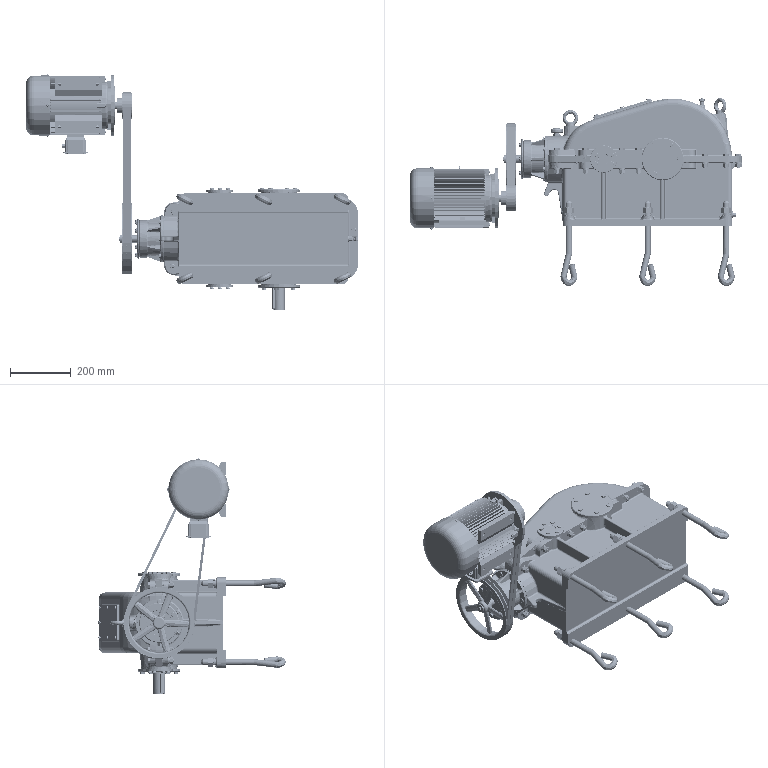Assembly | SolidWorks | mm | 166 component files | 167 solids | 7036 faces | box 1096.96 x 620.43 x 778.46 mm | volume 26160127 mm3 | plane 2138 | cone 2016 | cylinder 1637 | spline 832 | torus 356 | sphere 57 | commonest cylinder face diameters 8 x245 20 x128 324 x107 310.492 x106 6 x100 13.5 x78 10 x76 12 x74
Bill of materials:
BevelGear24_2.5 | 1 |  | Bevel-type pinion: a conical toothed body with a plain cylindrical hub on its back side and a through bore with one keyway.
BevelGear82_2.51 | 1 |  | Large, flat bevel-type gear: a wide disc with many fine teeth on a conical outer face, a flat central face, a small hub boss on the back and a keyed bore.
BreatherCap | 1 | Q235-A | Turned part with a mushroom-shaped head: a large domed, chamfered round head, a waisted neck, a hex section and a cylindrical spigot with a small axial bore.
Bushing0718 | 1 |  | Flanged, hollow, axisymmetric hub or housing: a large bolt flange between a short wide collar on one side and a long cylindrical barrel on the other, joined by gusset ribs, with a central through bore.
CylindricalGear106_3 | 1 |  | Spur gear with straight teeth: a thin, wide disc with many fine teeth, a recessed web with six lightening/through holes, a raised central hub and a keyed bore.
CylindricalGear24_3 | 1 |  | Spur gear with a long face width: straight teeth along a long cylindrical body and a through bore with one keyway.
Default | 1 |  | Envelope looks like a foot- and flange-mounted rotating machine, similar to an electric motor: a finned cylindrical body, a domed rear cover, a mounting foot, a front flange and a protruding plain shaft.
Gasket | 2 |  | Plain flat washer-like ring: a thin annular disc with a central round hole and parallel flat faces.
GB_T10708.3-1989TypeBRubberDustSealFB20_35_7 | 1 |  | Stepped ring: a rectangular-section annulus with a smaller-diameter, chamfered or tapered lip on one face, and a thin wall relative to its diameter.
GB_T10708.3-1989TypeBRubberDustSealFB45_65_8 | 1 |  | Wide, thin annular ring with a conical (tapered) inner bore and a short tapered shoulder below a flat-sided main band.
GB_T117-2000[TaperPin8_30] | 2 |  | Solid cylindrical pin with slightly domed/crowned ends on both sides; resembles a dowel-type pin.
Default | 4 |  | Rolling-element bearing-like assembly: concentric outer and inner rings with a single row of rolling elements between them; the inner ring sticks out axially past the outer ring on one side.
Default | 2 |  | Rolling-element bearing-like assembly with thinner section: outer and inner rings with one row of rolling elements; the inner ring sticks out axially on one side; larger bore relative to outer diameter than unnamed part.
GB_T41-2000HexNutType1C-gradeM20 | 6 |  | Hexagonal prism with a plain round through-bore, chamfered corners on both end faces; nut-like shape.
GB_T5780-2016[HexHeadBoltGradeCM12_80] | 8 |  | Hex-head bolt-like part with a long, plain cylindrical shank and chamfered tip.
GB_T5781-2000[HexHeadBoltFullThreadGradeCM12_40] | 5 |  | Hex-head bolt-like part with a medium-length plain cylindrical shank and chamfered tip.
GB_T5781-2000[HexHeadBoltFullThreadGradeCM6_16] | 8 |  | Short hex-head bolt-like part with a plain cylindrical shank, small fillet under the head and chamfered tip.
GB_T5781-2000[HexHeadBoltFullThreadGradeCM8_16] | 30 |  | Short hex-head bolt-like part with a plain shank, about 2x head width in length, and a chamfered tip.
GB_T5781-2000[HexHeadBoltFullThreadGradeCM8_20] | 6 |  | Short hex-head bolt-like part with a plain cylindrical shank and chamfered tip.
GB_T5781-2000HexHeadBoltFullThreadC-gradeM10_30 | 1 |  | Hex-head bolt-like part: hexagonal head with chamfered top edges, a thin cylindrical shoulder under the head, and a smooth cylindrical shank with a chamfered tip.
GB_T5781-2000HexHeadBoltFullThreadC-gradeM8_25 | 1 |  | Hex-head bolt-like part with a round washer-face flange under the head and a smooth cylindrical shank ending in a chamfered tip.
GB_T6170-2000[Type1HexNutGradeAAndBM12] | 13 |  | Hexagonal nut-like body with a central through bore and chamfered corners on both faces.
GB_T825-1988[LiftingEyeBoltM20] | 2 |  | Eye-shaped part: a toroidal ring loop on a cylindrical collar, with a plain cylindrical shank coming out of the collar.
GB_T93-1987[StandardSpringWasher(Assembly)12] | 13 |  | Flat annular ring with one narrow radial cut through the ring; the ends sit in the same plane.
GB_T93-1987StandardSpringWasher(Part)20_10 | 6 |  | Split annular ring with a rectangular section, twisted into one helical turn so the cut ends are offset along the axis; spring-lock-washer-like shape.
GB_T95-2002[FlatWasherGradeC12] | 13 |  | Plain flat annular disc (washer-like) with square edges and a central round hole.
GB_T97.2-1985FlatWasherChamferedTypeA-grade20_3 | 6 |  | Thin flat annular disc with a central round hole and a small chamfer on one outer edge.
HighSpeedAxisEndCoverA | 1 |  | Thin circular flange plate with six evenly spaced through-holes on a bolt circle and a central raised stepped cylindrical boss with a through-bore.
InputAxis | 1 |  | Stepped cylindrical shaft with several diameter sections, a larger central section, and one end face with a conical centre recess and a small slot or notch at the edge.
IntermediateAxis | 1 |  | Stepped cylindrical shaft with a thin raised collar ring partway along its length and a small notch at one end.
JB_ZQ4363-2006AnchorBoltTypeA20_630 | 6 |  | Bent round wire with a tight teardrop-shaped eye loop at one end, a short angled leg, and a long straight leg with a chamfered tip; cotter-pin-like or hook-like form.
JB_ZQ4450-1997[ExternalHexPlugM12_1.25] | 1 |  | Plug-like part: external hex drive, thin circular flange, undercut groove, and a chamfered cylindrical pilot/shank.
Key12-8-70 | 1 |  | Rectangular bar with fully rounded ends and slightly chamfered edges; parallel-key-like prism.
Key16-10-63 | 1 |  | Solid bar with rounded ends: a straight prism whose outline is a rectangle with two semicircular ends, with small chamfers on the edges. Moderately elongated, roughly 3.5:1 length to width in the rendered view.
Key6-6-25 | 1 |  | Short, stocky bar with rounded ends: a stadium-outline prism with chamfered edges, about 2.4:1 length to width, with height close to width.
Key6-6-32 | 1 |  | Bar with rounded ends: a stadium-outline prism with chamfered edges, about 3.2:1 length to width.
Key8-7-28 | 1 |  | Bar with rounded ends: a stadium-outline prism with chamfered edges, about 2.8:1 length to width, with a near-square cross-section.
Key8-7-40 | 1 |  | Long, slender bar with rounded ends: a stadium-outline prism with chamfered edges, about 5:1 length to width.
Key8-7-70 | 1 |  | Very slender bar with rounded ends: a stadium-outline prism with chamfered edges, about 7:1 length to width.
MachineBase | 1 |  | Open-top, box-shaped housing body. A rectangular wall shell is divided into compartments by internal ribs. The top has a perimeter flange interrupted by two semicircular cut-outs of different sizes, each with a bolt-hole pattern on the boss face. There are flanged ends with holes, extra holes on the side walls, and a hook-like lug on each end.
MachineCover | 1 |  | Hollow cover shell with an arched, sloping crown on top of a flat perimeter flange. The flange has two semicircular cut-outs of different sizes with small hole patterns, plus many perimeter holes. The top face has a rectangular opening ringed by small holes, and there are bosses or side protrusions on an end wall.
OilGauge | 1 |  | Long, thin, straight cylindrical rod or tube with a stepped head at one end. The head has a knurled or toothed outer cap, with concentric raised rings on its end face.
OutputAxis0717 | 1 |  | Stepped cylindrical shaft. Several diameters step down along its length, there is a thin raised collar near the middle, and keyway-like slots are cut into two of the diameter sections.
OutputAxisEndCover2-0717 | 1 |  | Solid circular cover disc with a chamfered outer edge and six through holes evenly spaced on a bolt circle. One face has a stepped, two-diameter spigot, with no central bore.
OutputAxisEndCover2-0718 | 1 |  | Flanged ring with a large central through bore. A wide chamfered base flange carries six evenly spaced through holes. A stepped intermediate ring and a raised cylindrical boss surround the bore.
SecondaryEndCover | 2 |  | Round, flat flange-like disc with six holes evenly spaced on a bolt circle. A circular feature sits at the center of the top face, and the underside steps down through a slightly smaller shoulder to a smaller cylindrical spigot.
SightHoleCoverA | 1 |  | Thin, flat rectangular plate with rounded corners and eight small round through holes around its edges.
V-beltL459x2 | 1 | Rubber | Closed teardrop- or pear-shaped loop made of a thin band, with a large rounded end, a small rounded end and two straight sides that taper between them. Edge views show two parallel bands side by side with a narrow gap between them.
A | 1 | Plain Carbon Steel | Spoked wheel with a twin-groove rim, resembling a two-groove V-belt pulley.
V-beltSmallSolidWheel86x24.075x48 | 1 | Plain Carbon Steel | Pulley-like body of revolution with two V-shaped circumferential grooves and a cylindrical hub on one side. A central through bore has a single rectangular keyway.
Mates:
1. concentric | OutputAxis0717-1 face at (-30, 0, 58.75) dir (0, 0, -1) r 27.5 | CylindricalGear106_3-1 face at (-30, 0, 35.75) dir (0, 0, 1) r 44
2. concentric | IntermediateAxis-1 face at (-225, 0, -13.099) dir (0, 0, 1) r 15 | CylindricalGear24_3-1 face at (-225, 0, 76.901) dir (0, 0, -1) r 15
3. concentric | IntermediateAxis-1 face at (-225, 0, -56.099) dir (0, 0, 1) r 15 | BevelGear82_2.51-1 face at (-225, 0, -6.098) dir (0, 0, -1) r 15
4. coincident | IntermediateAxis-1 face at (-225, 0, -23.099) dir (0, 0, -1) | BevelGear82_2.51-1 face at (-271.987, 53.409, -23.099) dir (0, 0, 1)
5. coincident | BevelGear82_2.51-1 sketch point at (-225, 0, 0) dir (1, 0, 0) | BevelGear24_2.5-1 sketch point at (-225, 0, 0) dir (1, 0, 0)
6. concentric | MachineBase-1 face at (200.001, 0, 0) dir (-1, 0, 0) r 54 | BevelGear24_2.5-1 face at (-357.363, 0, 0) dir (1, 0, 0) r 16
7. perpendicular | BevelGear82_2.51-1 face at (-227.438, 2.771, -56.098) dir (0, 0, -1) | BevelGear24_2.5-1 face at (-330.363, 2.308, -2.88) dir (-1, 0, 0)
8. concentric | InputAxis-1 face at (-297.364, 0, 0) dir (-1, 0, 0) r 10 | BevelGear24_2.5-1 face at (-357.363, 0, 0) dir (1, 0, 0) r 16
9. coincident | InputAxis-1 face at (-297.364, 0, 0) dir (1, 0, 0) | BevelGear24_2.5-1 face at (-297.364, 11.819, -14.749) dir (1, 0, 0)
10. concentric | MachineBase-1 face at (200.001, 0, 0) dir (-1, 0, 0) r 54 | Bushing0718-1 face at (-490, 0, 0) dir (-1, 0, 0) r 54
11. concentric | MachineBase-1 face at (-225, 0, -147) dir (0, 0, 1) r 26 | IntermediateAxis-1 face at (-225, 0, 61.901) dir (0, 0, 1) r 12.5
12. coincident | MachineBase-1 face at (-410, 0, 0) dir (-1, 0, 0) | Bushing0718-1 face at (-410, 38.5, -66.684) dir (1, 0, 0)
13. concentric | MachineBase-1 face at (-225, 0, -147) dir (0, 0, 1) r 26 | IntermediateAxis-1 face at (-225, 0, 61.901) dir (0, 0, 1) r 12.5
14. concentric | MachineBase-1 face at (-30, 0, -147) dir (0, 0, 1) r 45 | OutputAxis0717-1 face at (-30, 0, 107.25) dir (0, 0, -1) r 25
15. concentric | OutputAxis0717-1 face at (-30, 0, 107.25) dir (0, 0, -1) r 25 | GB_T297-94TaperedRollerBearing30210-0717-1 face at (-30, 0, 109) dir (0, 0, 1) r 25
16. coincident | OutputAxis0717-1 face at (-30, 0, 107.25) dir (0, 0, 1) | GB_T297-94TaperedRollerBearing30210-0717-1 face at (-27.138, 32.397, 107.25) dir (0, 0, 1)
17. concentric | OutputAxis0717-1 face at (-30, 0, -67.75) dir (0, 0, -1) r 25 | GB_T297-94TaperedRollerBearing30210-0717-2 face at (-30, 0, -104.5) dir (0, 0, -1) r 25
18. coincident | MachineBase-1 face at (0, 0, 92) dir (0, 0, -1) | GB_T297-94TaperedRollerBearing30210-0717-1 face at (-26.041, 44.825, 92) dir (0, 0, -1)
19. coincident | OutputAxis0717-1 face at (-30, 0, -102.75) dir (0, 0, -1) | GB_T297-94TaperedRollerBearing30210-0717-2 face at (-25.034, 32.142, -102.75) dir (0, 0, -1)
20. concentric | MachineBase-1 face at (-30, 0, -147) dir (0, 0, 1) r 45 | OutputAxisEndCover2-0717-1 face at (-30, 0, 147) dir (0, 0, 1) r 70
21. concentric | IntermediateAxis-1 face at (-225, 0, 61.901) dir (0, 0, 1) r 12.5 | GB_T297-94TaperedRollerBearing30205-1 face at (-225, 0, 104.151) dir (0, 0, 1) r 26
22. coincident | IntermediateAxis-1 face at (-225, 0, 102.901) dir (0, 0, 1) | GB_T297-94TaperedRollerBearing30205-1 face at (-225, 17.34, 102.901) dir (0, 0, 1)
23. concentric | MachineBase-1 face at (-225, 0, -147) dir (0, 0, 1) r 26 | SecondaryEndCover-1 face at (-225, 0, 147) dir (0, 0, 1) r 45
24. coincident | MachineBase-1 face at (-225, 0, 147) dir (0, 0, 1) | SecondaryEndCover-1 face at (-225, 40, 147) dir (0, 0, -1)
25. coincident | MachineBase-1 face at (-30, 0, 147) dir (0, 0, 1) | OutputAxisEndCover2-0717-1 face at (-0.9949, 52.523, 147) dir (0, 0, -1)
26. concentric | MachineBase-1 face at (-225, 0, -147) dir (0, 0, 1) r 26 | SecondaryEndCover-2 face at (-225, 0, -147) dir (0, 0, -1) r 45
27. coincident | MachineBase-1 face at (-225, 0, -147) dir (0, 0, -1) | SecondaryEndCover-2 face at (-225, 40, -147) dir (0, 0, 1)
28. concentric | MachineBase-1 face at (-30, 0, -147) dir (0, 0, 1) r 45 | OutputAxisEndCover2-0718-1 face at (-30, 0, -147) dir (0, 0, -1) r 70
29. coincident | MachineBase-1 face at (-30, 0, -147) dir (0, 0, -1) | OutputAxisEndCover2-0718-1 face at (-30, 60, -147) dir (0, 0, 1)
30. coincident | SightHoleCoverA-1 face at (-162.617, 165.059, 0) dir (0.2889, -0.9574, 0) | MachineCover-1 face at (-71.668, 192.504, -55) dir (-0.2889, 0.9574, 0)
31. concentric | SightHoleCoverA-1 face at (-76.455, 191.059, 0) dir (0.2889, -0.9574, 0) r 3.25 | MachineCover-1 face at (-76.455, 191.059, 0) dir (-0.2889, 0.9574, 0) r 3
32. concentric | SightHoleCoverA-1 face at (-248.78, 139.059, 0) dir (0.2889, -0.9574, 0) r 3.25 | MachineCover-1 face at (-248.78, 139.059, 0) dir (-0.2889, 0.9574, 0) r 3
33. coincident | MachineBase-1 face at (-360, 0, 100) dir (0, 1, 0) | MachineCover-1 face at (-360, 0, 100) dir (0, -1, 0)
34. concentric | OutputAxis0717-1 face at (-30, 0, 107.25) dir (0, 0, -1) r 25 | MachineCover-1 face at (-30, 0, -147) dir (0, 0, 1) r 45
35. concentric | MachineBase-1 face at (180, 0, 125) dir (0, 1, 0) r 6.75 | MachineCover-1 face at (180, 0, 125) dir (0, -1, 0) r 6.75
36. concentric | MachineBase-1 face at (180, 0, -125) dir (0, 1, 0) r 6.75 | MachineCover-1 face at (180, 0, -125) dir (0, -1, 0) r 6.75
37. concentric | MachineBase-1 face at (-380, 0, 90) dir (0, 1, 0) r 6.75 | MachineCover-1 face at (-380, 0, 90) dir (0, -1, 0) r 6.75
38. concentric | GB_T5781-2000[HexHeadBoltFullThreadGradeCM6_16]-1 face at (-251.091, 146.718, -50) dir (0.2889, -0.9574, 0) r 3 | SightHoleCoverA-1 face at (-248.78, 139.059, -50) dir (0.2889, -0.9574, 0) r 3.25
39. coincident | GB_T5781-2000[HexHeadBoltFullThreadGradeCM6_16]-1 face at (-244.408, 144.557, -50) dir (0.2889, -0.9574, 0) | SightHoleCoverA-1 face at (-163.773, 168.889, 0) dir (-0.2889, 0.9574, 0)
40. concentric | Bushing0718-1 face at (-347, 32.5, -56.292) dir (-1, 0, 0) r 4.5 | GB_T5781-2000[HexHeadBoltFullThreadGradeCM8_20]-1 face at (-425.3, 32.5, -56.292) dir (1, 0, 0) r 4
41. coincident | Bushing0718-1 face at (-420, 27, -46.765) dir (-1, 0, 0) | GB_T5781-2000[HexHeadBoltFullThreadGradeCM8_20]-1 face at (-420, 39.146, -52.803) dir (1, 0, 0)
42. concentric | InputAxis-1 face at (-465.364, 0, 0) dir (-1, 0, 0) r 12.5 | GB_T297-94TaperedRollerBearing30205-3 face at (-466.614, 0, 0) dir (-1, 0, 0) r 12.5
43. coincident | InputAxis-1 face at (-450.364, 0, 0) dir (-1, 0, 0) | GB_T297-94TaperedRollerBearing30205-3 face at (-450.364, 18.954, 0) dir (1, 0, 0)
44. concentric | InputAxis-1 face at (-297.364, 0, 0) dir (-1, 0, 0) r 10 | GB_T297-94TaperedRollerBearing30205-4 face at (-356.114, 0, 0) dir (1, 0, 0) r 12.5
45. coincident | InputAxis-1 face at (-372.364, 0, 0) dir (1, 0, 0) | GB_T297-94TaperedRollerBearing30205-4 face at (-372.364, 18.954, 0) dir (-1, 0, 0)
46. concentric | IntermediateAxis-1 face at (-225, 0, -115.099) dir (0, 0, 1) r 12.5 | GB_T297-94TaperedRollerBearing30205-2 face at (-225, 0, -108.25) dir (0, 0, -1) r 26
47. coincident | MachineBase-1 face at (0, 0, -92) dir (0, 0, 1) | GB_T297-94TaperedRollerBearing30205-2 face at (-225, 18.954, -92) dir (0, 0, 1)
48. concentric | Bushing0718-1 face at (-490, 0, 0) dir (-1, 0, 0) r 62 | HighSpeedAxisEndCoverA-1 face at (-484, 0, 0) dir (-1, 0, 0) r 66
49. coincident | Bushing0718-1 face at (-490, 13, -22.517) dir (-1, 0, 0) | HighSpeedAxisEndCoverA-1 face at (-490, 57.158, 33) dir (1, 0, 0)
50. concentric | Bushing0718-1 face at (-490, 46.765, -27) dir (-1, 0, 0) r 4 | HighSpeedAxisEndCoverA-1 face at (-498, 46.765, -27) dir (-1, 0, 0) r 4.5
51. concentric | Bushing0718-1 face at (-490, 46.765, 27) dir (-1, 0, 0) r 4 | HighSpeedAxisEndCoverA-1 face at (-498, 46.765, 27) dir (-1, 0, 0) r 4.5
52. concentric | HighSpeedAxisEndCoverA-1 face at (-498, -46.765, 27) dir (-1, 0, 0) r 4.5 | GB_T5781-2000[HexHeadBoltFullThreadGradeCM8_16]-1 face at (-503.3, -46.765, 27) dir (1, 0, 0) r 4
53. coincident | HighSpeedAxisEndCoverA-1 face at (-498, 0, 0) dir (-1, 0, 0) | GB_T5781-2000[HexHeadBoltFullThreadGradeCM8_16]-1 face at (-498, -41.157, 31.987) dir (1, 0, 0)
54. concentric | InputAxis-1 face at (-515.364, 0, 0) dir (-1, 0, 0) r 10 | V-beltLargeEllipticalSpokeWheel235x52.875x331-1 face at (-550.57, 0, 0) dir (-1, 0, 0) r 10
55. coincident | InputAxis-1 face at (-515.364, 0, 0) dir (-1, 0, 0) | V-beltLargeEllipticalSpokeWheel235x52.875x331-1 face at (-515.364, 12.507, -15.607) dir (1, 0, 0)
56. parallel | V-beltSmallSolidWheel86x24.075x48-1 face at (-548.364, -87, 440.206) dir (-1, 0, 0) | V-beltLargeEllipticalSpokeWheel235x52.875x331-1 face at (-548.364, 62.566, -78.074) dir (-1, 0, 0)
57. concentric | V-beltLargeEllipticalSpokeWheel235x52.875x331-1 face at (-539.364, 0, 0) dir (-1, 0, 0) r 106.05 | V-beltL459x2-1 face at (-539.364, 0, 0) dir (-1, 0, 0) r 109.938
58. concentric | V-beltSmallSolidWheel86x24.075x48-1 face at (-539.364, -130, 440.206) dir (1, 0, 0) r 31.55 | V-beltL459x2-1 face at (-539.364, -130, 440.206) dir (1, 0, 0) r 35.438
59. concentric | MachineCover-1 face at (-380, 0, 90) dir (0, -1, 0) r 6.75 | GB_T5780-2016[HexHeadBoltGradeCM12_80]-1 face at (-380, 37.5, 90) dir (0, -1, 0) r 6
60. coincident | MachineCover-1 face at (-376, 30, 87.854) dir (0, 1, 0) | GB_T5780-2016[HexHeadBoltGradeCM12_80]-1 face at (-369.608, 30, 90) dir (0, -1, 0)
61. concentric | GB_T5780-2016[HexHeadBoltGradeCM12_80]-1 face at (-380, 37.5, 90) dir (0, -1, 0) r 6 | GB_T95-2002[FlatWasherGradeC12]-1 face at (-380, -41.145, 90) dir (0, -1, 0) r 6.75
62. coincident | MachineBase-1 face at (-305.467, -30, 140) dir (0, -1, 0) | GB_T95-2002[FlatWasherGradeC12]-1 face at (-386.75, -30, 90) dir (0, 1, 0)
63. concentric | GB_T5780-2016[HexHeadBoltGradeCM12_80]-1 face at (-380, 37.5, 90) dir (0, -1, 0) r 6 | GB_T93-1987[StandardSpringWasher(Assembly)12]-1 face at (-380, -35.6, 90) dir (0, 1, 0) r 6.1
64. coincident | GB_T95-2002[FlatWasherGradeC12]-1 face at (-386.75, -32.5, 90) dir (0, -1, 0) | GB_T93-1987[StandardSpringWasher(Assembly)12]-1 face at (-380, -32.5, 90) dir (0, 1, 0)
65. concentric | GB_T5780-2016[HexHeadBoltGradeCM12_80]-1 face at (-380, 37.5, 90) dir (0, -1, 0) r 6 | GB_T6170-2000[Type1HexNutGradeAAndBM12]-1 face at (-380, -46.4, 90) dir (0, 1, 0) r 6
66. coincident | GB_T93-1987[StandardSpringWasher(Assembly)12]-1 face at (-380, -35.6, 90) dir (0, -1, 0) | GB_T6170-2000[Type1HexNutGradeAAndBM12]-1 face at (-389, -35.6, 105.588) dir (0, 1, 0)
67. coincident | MachineCover-1 face at (182, 10, -84.323) dir (0, 1, 0) | GB_T117-2000[TaperPin8_30]-2 edge at (220, 10, 0) dir (0, -1, 0) r 4.138
68. concentric | MachineCover-1 face at (-285, 0, 125) dir (0, -1, 0) r 6.75 | GB_T5780-2016[HexHeadBoltGradeCM12_80]-3 face at (-285, 37.5, 125) dir (0, -1, 0) r 6
69. coincident | MachineCover-1 face at (-306.888, 30, 140) dir (0, 1, 0) | GB_T5780-2016[HexHeadBoltGradeCM12_80]-3 face at (-274.608, 30, 125) dir (0, -1, 0)
70. concentric | GB_T5780-2016[HexHeadBoltGradeCM12_80]-3 face at (-285, 37.5, 125) dir (0, -1, 0) r 6 | GB_T95-2002[FlatWasherGradeC12]-3 face at (-285, -41.145, 125) dir (0, -1, 0) r 12
71. concentric | GB_T5780-2016[HexHeadBoltGradeCM12_80]-3 face at (-285, 37.5, 125) dir (0, -1, 0) r 6 | GB_T93-1987[StandardSpringWasher(Assembly)12]-3 face at (-285, -32.5, 125) dir (0, -1, 0) r 9.183
72. coincident | MachineBase-1 face at (-305.467, -30, 140) dir (0, -1, 0) | GB_T95-2002[FlatWasherGradeC12]-3 face at (-291.75, -30, 125) dir (0, 1, 0)
73. coincident | GB_T95-2002[FlatWasherGradeC12]-3 face at (-291.75, -32.5, 125) dir (0, -1, 0) | GB_T93-1987[StandardSpringWasher(Assembly)12]-3 face at (-285, -32.5, 125) dir (0, 1, 0)
74. concentric | GB_T5780-2016[HexHeadBoltGradeCM12_80]-3 face at (-285, 37.5, 125) dir (0, -1, 0) r 6 | GB_T6170-2000[Type1HexNutGradeAAndBM12]-3 face at (-285, -46.4, 125) dir (0, 1, 0) r 6
75. coincident | GB_T93-1987[StandardSpringWasher(Assembly)12]-3 face at (-285, -35.6, 125) dir (0, -1, 0) | GB_T6170-2000[Type1HexNutGradeAAndBM12]-3 face at (-294, -35.6, 140.588) dir (0, 1, 0)
76. concentric | MachineCover-1 face at (110, 0, 125) dir (0, -1, 0) r 6.75 | GB_T5781-2000[HexHeadBoltFullThreadGradeCM12_40]-1 face at (110, 17.5, 125) dir (0, -1, 0) r 6
77. coincident | MachineCover-1 face at (182, 10, -84.323) dir (0, 1, 0) | GB_T5781-2000[HexHeadBoltFullThreadGradeCM12_40]-1 face at (120.392, 10, 125) dir (0, -1, 0)
78. concentric | GB_T5781-2000[HexHeadBoltFullThreadGradeCM12_40]-1 face at (110, 17.5, 125) dir (0, -1, 0) r 6 | GB_T95-2002[FlatWasherGradeC12]-6 face at (110, -21.145, 125) dir (0, -1, 0) r 12
79. coincident | MachineBase-1 face at (182, -10, -84.323) dir (0, -1, 0) | GB_T95-2002[FlatWasherGradeC12]-6 face at (103.25, -10, 125) dir (0, 1, 0)
80. concentric | GB_T5781-2000[HexHeadBoltFullThreadGradeCM12_40]-1 face at (110, 17.5, 125) dir (0, -1, 0) r 6 | GB_T93-1987[StandardSpringWasher(Assembly)12]-6 face at (110, -12.5, 125) dir (0, -1, 0) r 9.183
81. coincident | GB_T95-2002[FlatWasherGradeC12]-6 face at (103.25, -12.5, 125) dir (0, -1, 0) | GB_T93-1987[StandardSpringWasher(Assembly)12]-6 face at (110, -12.5, 125) dir (0, 1, 0)
82. concentric | GB_T5781-2000[HexHeadBoltFullThreadGradeCM12_40]-1 face at (110, 17.5, 125) dir (0, -1, 0) r 6 | GB_T6170-2000[Type1HexNutGradeAAndBM12]-6 face at (110, -26.4, 125) dir (0, 1, 0) r 6
83. coincident | GB_T93-1987[StandardSpringWasher(Assembly)12]-6 face at (110, -15.6, 125) dir (0, -1, 0) | GB_T6170-2000[Type1HexNutGradeAAndBM12]-6 face at (125.588, -15.6, 116) dir (0, 1, 0)
84. concentric | MachineCover-1 face at (220, 0, 30) dir (0, -1, 0) r 6.75 | GB_T5781-2000[HexHeadBoltFullThreadGradeCM12_40]-4 face at (220, 17.5, 30) dir (0, -1, 0) r 6
85. coincident | MachineCover-1 face at (182, 10, -84.323) dir (0, 1, 0) | GB_T5781-2000[HexHeadBoltFullThreadGradeCM12_40]-4 face at (230.079, 10, 32.534) dir (0, -1, 0)
86. concentric | GB_T5781-2000[HexHeadBoltFullThreadGradeCM12_40]-4 face at (220, 17.5, 30) dir (0, -1, 0) r 6 | GB_T95-2002[FlatWasherGradeC12]-8 face at (220, -21.145, 30) dir (0, -1, 0) r 12
87. concentric | GB_T5781-2000[HexHeadBoltFullThreadGradeCM12_40]-4 face at (220, 17.5, 30) dir (0, -1, 0) r 6 | GB_T93-1987[StandardSpringWasher(Assembly)12]-8 face at (220, -12.5, 30) dir (0, -1, 0) r 9.183
88. coincident | MachineBase-1 face at (182, -10, -84.323) dir (0, -1, 0) | GB_T95-2002[FlatWasherGradeC12]-8 face at (213.25, -10, 30) dir (0, 1, 0)
89. coincident | GB_T95-2002[FlatWasherGradeC12]-8 face at (213.25, -12.5, 30) dir (0, -1, 0) | GB_T93-1987[StandardSpringWasher(Assembly)12]-8 face at (220, -12.5, 30) dir (0, 1, 0)
90. concentric | GB_T5781-2000[HexHeadBoltFullThreadGradeCM12_40]-4 face at (220, 17.5, 30) dir (0, -1, 0) r 6 | GB_T6170-2000[Type1HexNutGradeAAndBM12]-8 face at (220, -26.4, 30) dir (0, 1, 0) r 6
91. coincident | GB_T93-1987[StandardSpringWasher(Assembly)12]-8 face at (220, -15.6, 30) dir (0, -1, 0) | GB_T6170-2000[Type1HexNutGradeAAndBM12]-8 face at (235.588, -15.6, 21) dir (0, 1, 0)
92. concentric | OutputAxisEndCover2-0717-1 face at (-58.402, 47.099, 163) dir (0, 0, 1) r 4.5 | GB_T5781-2000[HexHeadBoltFullThreadGradeCM8_16]-7 face at (-58.402, 47.099, 168.3) dir (0, 0, -1) r 4
93. coincident | OutputAxisEndCover2-0717-1 face at (-30, 0, 163) dir (0, 0, 1) | GB_T5781-2000[HexHeadBoltFullThreadGradeCM8_16]-7 face at (-58.402, 54.605, 163) dir (0, 0, -1)
94. concentric | SecondaryEndCover-1 face at (-225, 30.5, 161) dir (0, 0, 1) r 4.5 | GB_T5781-2000[HexHeadBoltFullThreadGradeCM8_16]-13 face at (-225, 30.5, 166.3) dir (0, 0, -1) r 4
95. coincident | SecondaryEndCover-1 face at (-225, 0, 161) dir (0, 0, 1) | GB_T5781-2000[HexHeadBoltFullThreadGradeCM8_16]-13 face at (-225, 38.006, 161) dir (0, 0, -1)
96. concentric | SecondaryEndCover-2 face at (-251.414, -15.25, -161) dir (0, 0, -1) r 4.5 | GB_T5781-2000[HexHeadBoltFullThreadGradeCM8_16]-19 face at (-251.414, -15.25, -166.3) dir (0, 0, 1) r 4
97. coincident | SecondaryEndCover-2 face at (-225, 0, -161) dir (0, 0, -1) | GB_T5781-2000[HexHeadBoltFullThreadGradeCM8_16]-19 face at (-251.414, -7.744, -161) dir (0, 0, 1)
98. concentric | OutputAxisEndCover2-0718-1 face at (-30, 55, -163) dir (0, 0, -1) r 4.5 | GB_T5781-2000[HexHeadBoltFullThreadGradeCM8_16]-26 face at (-30, 55, -168.3) dir (0, 0, 1) r 4
99. coincident | OutputAxisEndCover2-0718-1 face at (-30, 0, -163) dir (0, 0, -1) | GB_T5781-2000[HexHeadBoltFullThreadGradeCM8_16]-26 face at (-30, 62.506, -163) dir (0, 0, 1)
100. concentric | MachineCover-1 face at (-380, 75, 0) dir (0, 1, 0) r 9 | BreatherCap-1 face at (-380, 103, 0) dir (0, 1, 0) r 9
101. coincident | MachineCover-1 face at (-380, 75, 0) dir (0, 1, 0) | BreatherCap-1 face at (-372.3, 75, 0) dir (0, -1, 0)
102. concentric | MachineCover-1 face at (100, 180, -50) dir (0, 1, 0) r 6 | OilGauge-1 face at (100, -180, -50) dir (0, 1, 0) r 3
103. coincident | MachineCover-1 face at (100, 180, -50) dir (0, 1, 0) | OilGauge-1 face at (104.5, 180, -50) dir (0, -1, 0)
104. concentric | MachineBase-1 face at (200, -184, 0) dir (1, 0, 0) r 6 | JB_ZQ4450-1997[ExternalHexPlugM12_1.25]-1 face at (212, -184, 0) dir (1, 0, 0) r 6
105. coincident | MachineBase-1 face at (200, 0, 100) dir (1, 0, 0) | JB_ZQ4450-1997[ExternalHexPlugM12_1.25]-1 face at (200, -171, 0.06629) dir (-1, 0, 0)
106. concentric | MachineCover-1 face at (-335, 110, 0) dir (0, 1, 0) r 10 | GB_T825-1988[LiftingEyeBoltM20]-1 face at (-335, 110, 0) dir (0, 1, 0) r 10
107. coincident | MachineCover-1 face at (-335, 110, 0) dir (0, 1, 0) | GB_T825-1988[LiftingEyeBoltM20]-1 face at (-335, 110, 0) dir (0, -1, 0)
108. concentric | MachineCover-1 face at (160, 150, 0) dir (0, 1, 0) r 10 | GB_T825-1988[LiftingEyeBoltM20]-2 face at (160, 150, 0) dir (0, 1, 0) r 10
109. coincident | MachineCover-1 face at (160, 150, 0) dir (0, 1, 0) | GB_T825-1988[LiftingEyeBoltM20]-2 face at (160, 150, 0) dir (0, -1, 0)
110. concentric | MachineBase-1 face at (-340, -192, 130) dir (0, 1, 0) r 11 | JB_ZQ4363-2006AnchorBoltTypeA20_630-1 face at (-340, -138.83, 130) dir (0, -1, 0) r 10
111. concentric | JB_ZQ4363-2006AnchorBoltTypeA20_630-1 face at (-340, -138.83, 130) dir (0, -1, 0) r 10 | GB_T97.2-1985FlatWasherChamferedTypeA-grade20_3-1 face at (-340, -200.645, 130) dir (0, -1, 0) r 18.5
112. coincident | MachineBase-1 face at (-340, -192, 130) dir (0, 1, 0) | GB_T97.2-1985FlatWasherChamferedTypeA-grade20_3-1 face at (-350.5, -192, 130) dir (0, -1, 0)
113. concentric | JB_ZQ4363-2006AnchorBoltTypeA20_630-1 face at (-340, -138.83, 130) dir (0, -1, 0) r 10 | GB_T93-1987StandardSpringWasher(Part)20_10-1 sketch segment at (-340, -183.818, 130) dir (0, -1, 0) r 8.24
114. concentric | JB_ZQ4363-2006AnchorBoltTypeA20_630-1 face at (-340, -138.83, 130) dir (0, -1, 0) r 10 | GB_T41-2000HexNutType1C-gradeM20-1 face at (-340, -179.134, 130) dir (0, 1, 0) r 10
115. concentric | V-beltSmallSolidWheel86x24.075x48-1 face at (-524.364, -130, 440.206) dir (1, 0, 0) r 24.075 | FlangedMotorWithBase90L-1 face at (-522.956, -130, 440.206) dir (1, 0, 0) r 12
116. coincident | MachineBase-1 face at (500.666, -220, 90) dir (0, -1, 0) | FlangedMotorWithBase90L-1 face at (-811.676, -220, 490.206) dir (0, -1, 0)
117. parallel | V-beltSmallSolidWheel86x24.075x48-1 face at (-565.364, -118.686, 436.206) dir (0, 0, 1) | FlangedMotorWithBase90L-1 face at (-522.956, -118, 436.206) dir (0, 0, 1)
118. coincident | FlangedMotorWithBase90L-1 face at (-522.956, -118, 444.206) dir (0, 0, -1) | Key8-7-40-1 face at (-526.976, -115, 444.206) dir (0, 0, 1)
119. coincident | FlangedMotorWithBase90L-1 face at (-522.956, -122, 444.206) dir (0, 1, 0) | Key8-7-40-1 face at (-526.976, -122, 440.206) dir (0, -1, 0)
120. parallel | InputAxis-1 face at (-520.364, 5.788, -12.021) dir (0, 0.7803, 0.6253) | V-beltLargeEllipticalSpokeWheel235x52.875x331-1 face at (-515.364, 3.624, -9.32) dir (0, 0.7803, 0.6253)
121. coincident | InputAxis-1 face at (-329.364, 10.596, -8.425) dir (0, -0.7803, -0.6253) | BevelGear24_2.5-1 face at (-288.363, 10.345, -8.112) dir (0, -0.7803, -0.6253)
122. coincident | InputAxis-1 face at (-329.364, 5.913, -12.177) dir (0, 0.7803, 0.6253) | Key6-6-32-1 face at (-320.42, 5.663, -11.865) dir (0, -0.7803, -0.6253)
123. coincident | InputAxis-1 face at (-329.364, 6.593, -3.43) dir (0, 0.6253, -0.7803) | Key6-6-32-1 face at (-300.42, 4.252, -5.306) dir (0, -0.6253, 0.7803)
124. coincident | IntermediateAxis-1 face at (-240.421, 11.473, -27.699) dir (0.7508, 0.6605, 0) | BevelGear82_2.51-1 face at (-240.421, 11.473, -18.098) dir (0.7508, 0.6605, 0)
125. coincident | IntermediateAxis-1 face at (-229.395, 11.051, -27.699) dir (-0.6605, 0.7508, 0) | Key8-7-28-1 face at (-232.398, 8.409, -31.748) dir (0.6605, -0.7508, 0)
126. coincident | IntermediateAxis-1 face at (-240.421, 11.473, -27.699) dir (0.7508, 0.6605, 0) | Key8-7-28-1 face at (-240.025, 11.023, -31.748) dir (-0.7508, -0.6605, 0)
127. coincident | IntermediateAxis-1 face at (-234.415, 16.757, -8.499) dir (-0.7508, -0.6605, 0) | CylindricalGear24_3-1 face at (-234.018, 16.307, 66.901) dir (-0.7508, -0.6605, 0)
128. coincident | IntermediateAxis-1 face at (-235.401, 5.767, -8.499) dir (-0.6605, 0.7508, 0) | Key8-7-70-1 face at (-232.398, 8.409, 57.881) dir (0.6605, -0.7508, 0)
129. coincident | IntermediateAxis-1 face at (-240.421, 11.473, -8.499) dir (0.7508, 0.6605, 0) | Key8-7-70-1 face at (-240.025, 11.023, 57.881) dir (-0.7508, -0.6605, 0)
130. coincident | OutputAxis0717-1 face at (-62.89, -9.547, -4.65) dir (0.4954, -0.8687, 0) | CylindricalGear106_3-1 face at (-62.195, -9.151, 71.75) dir (0.4954, -0.8687, 0)
131. coincident | CylindricalGear106_3-1 face at (-62.195, -9.151, 71.75) dir (0.8687, 0.4954, 0) | Key16-10-63-1 face at (-58.232, -16.1, 3.729) dir (-0.8687, -0.4954, 0)
132. coincident | CylindricalGear106_3-1 face at (-54.269, -23.05, 71.75) dir (-0.4954, 0.8687, 0) | Key16-10-63-1 face at (-45.582, -18.096, 3.729) dir (0.4954, -0.8687, 0)
133. coincident | OutputAxis0717-1 face at (-46.697, -2.615, -163.75) dir (-0.8687, -0.4954, 0) | Key12-8-70-1 face at (-43.725, -7.827, -169.75) dir (0.8687, 0.4954, 0)
134. coincident | OutputAxis0717-1 face at (-48.049, -17.201, -163.75) dir (-0.4954, 0.8687, 0) | Key12-8-70-1 face at (-40.753, -13.039, -227.75) dir (0.4954, -0.8687, 0)
135. concentric | OutputAxis0717-1 face at (-30, 0, -169.75) dir (0.8687, 0.4954, 0) r 6 | Key12-8-70-1 face at (-43.725, -7.827, -169.75) dir (-0.8687, -0.4954, 0) r 6
136. concentric | InputAxis-1 face at (-297.364, 0, 0) dir (1, 0, 0) r 5 | Gasket-1 face at (-292.364, 0, 0) dir (-1, 0, 0) r 5.5
137. coincident | InputAxis-1 face at (-297.364, 0, 0) dir (1, 0, 0) | Gasket-1 face at (-297.364, 0, 0) dir (-1, 0, 0)
138. concentric | InputAxis-1 face at (-297.364, 0, 0) dir (1, 0, 0) r 5 | GB_T5781-2000HexHeadBoltFullThreadC-gradeM10_30-1 face at (-285.964, 0, 0) dir (1, 0, 0) r 5
139. coincident | Gasket-1 face at (-292.364, 0, 0) dir (1, 0, 0) | GB_T5781-2000HexHeadBoltFullThreadC-gradeM10_30-1 face at (-292.364, -9.233, 0.3031) dir (-1, 0, 0)
140. coincident | V-beltLargeEllipticalSpokeWheel235x52.875x331-1 face at (-548.364, 12.507, -15.607) dir (-1, 0, 0) | Gasket-2 face at (-548.364, 0, 0) dir (1, 0, 0)
141. concentric | InputAxis-1 face at (-545.364, 0, 0) dir (-1, 0, 0) r 4 | Gasket-2 face at (-548.364, 0, 0) dir (-1, 0, 0) r 5.5
142. coincident | Gasket-2 face at (-553.364, 0, 0) dir (-1, 0, 0) | GB_T5781-2000HexHeadBoltFullThreadC-gradeM8_25-1 face at (-553.364, 7.502, -0.2462) dir (1, 0, 0)
143. concentric | Gasket-2 face at (-548.364, 0, 0) dir (-1, 0, 0) r 5.5 | GB_T5781-2000HexHeadBoltFullThreadC-gradeM8_25-1 face at (-558.664, 0, 0) dir (-1, 0, 0) r 4
144. coincident | InputAxis-1 face at (-520.364, 2.036, -7.338) dir (0, 0.6253, -0.7803) | Key6-6-25-2 face at (-531.299, 4.377, -5.462) dir (0, -0.6253, 0.7803)
145. coincident | InputAxis-1 face at (-520.364, 10.471, -8.269) dir (0, -0.7803, -0.6253) | Key6-6-25-2 face at (-531.299, 10.471, -8.269) dir (0, 0.7803, 0.6253)
146. concentric | OutputAxis0717-1 face at (-30, 0, -102.75) dir (0, 0, -1) r 22.5 | GB_T10708.3-1989TypeBRubberDustSealFB45_65_8-1 face at (-30, 0, -104.5) dir (0, 0, 1) r 32.5
147. coincident | GB_T297-94TaperedRollerBearing30210-0717-2 face at (-23.129, 44.472, -104.5) dir (0, 0, -1) | GB_T10708.3-1989TypeBRubberDustSealFB45_65_8-1 face at (-15.237, 28.953, -104.5) dir (0, 0, 1)
148. concentric | InputAxis-1 face at (-465.364, 0, 0) dir (-1, 0, 0) r 12.5 | GB_T10708.3-1989TypeBRubberDustSealFB20_35_7-1 face at (-465.364, 0, 0) dir (1, 0, 0) r 17.5
149. coincident | GB_T10708.3-1989TypeBRubberDustSealFB20_35_7-1 face at (-465.364, -3.365, 17.173) dir (1, 0, 0) | GB_T297-94TaperedRollerBearing30205-3 face at (-465.364, 17.34, 0) dir (-1, 0, 0)
150. coincident | OutputAxis0717-1 face at (-30, 0, -11.25) dir (0, 0, 1) | CylindricalGear106_3-1 face at (-30, 0, -11.25) dir (0, 0, -1)
151. coincident | IntermediateAxis-1 face at (-225, 0, -13.099) dir (0, 0, 1) | CylindricalGear24_3-1 face at (-225, 0, -13.099) dir (0, 0, -1)
152. concentric | MachineCover-1 face at (-315, 0, 125) dir (0, -1, 0) r 4.936 | GB_T117-2000[TaperPin8_30]-1 face at (-315, -14.061, 125) dir (0, -1, 0) r 4.936
153. concentric | MachineCover-1 face at (220, 0, 0) dir (0, -1, 0) r 4.936 | GB_T117-2000[TaperPin8_30]-2 face at (220, -18, 0) dir (0, -1, 0) r 4.936
154. concentric | MachineCover-1 face at (-410, 65, 0) dir (-1, 0, 0) r 4 | GB_T5781-2000[HexHeadBoltFullThreadGradeCM8_20]-6 face at (-425.3, 65, 0) dir (1, 0, 0) r 4
155. coincident | V-beltLargeEllipticalSpokeWheel235x52.875x331-1 plane at (-539.364, 0, 0) dir (1, 0, 0) | V-beltL459x2-1 plane at (-539.364, 0, 0) dir (1, 0, 0)